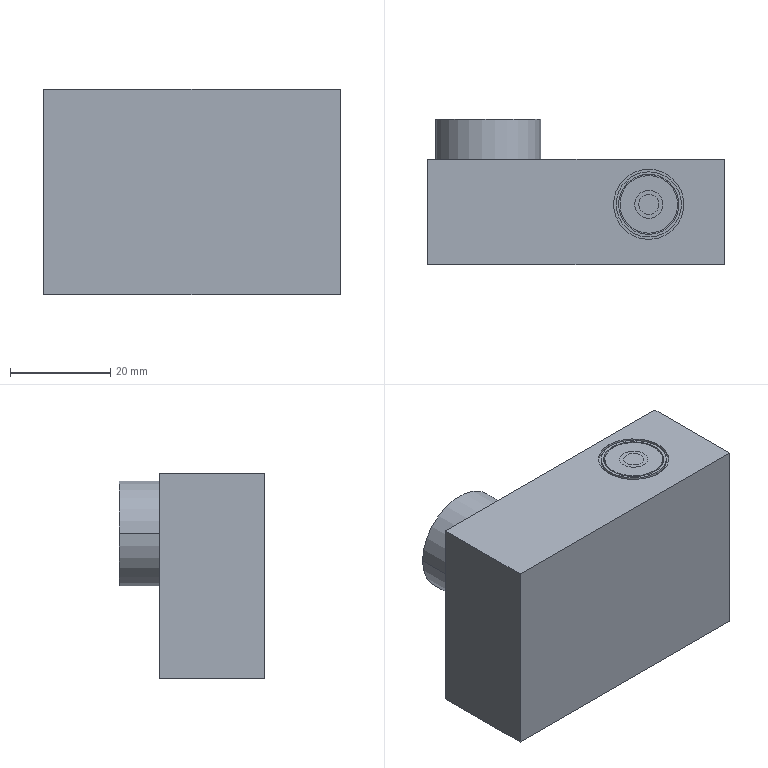Component | SolidWorks | Camera-1 | 1 solid | 38 faces | box 59 x 29 x 41 mm | volume 53051 mm3 | plane 18 | cylinder 14 | cone 4 | sphere 2 | commonest cylinder face diameters 11.5 x2 12 x2 14 x2 13 x2 17.5 x2 18.5 x2 21 x2
build123d program:
from build123d import *

# Parameters (mm, degrees)
SKETCH1_W           = 59
SKETCH1_H           = 41
BOSS_EXTRUDE1_DEPTH = 21
SKETCH5_R           = 7
SKETCH5_R_2         = 6.5
SKETCH5_R_3         = 6
SKETCH5_R_4         = 5.75
CUT_EXTRUDE1_DEPTH  = 0.5
SKETCH6_R           = 6
SKETCH6_R_2         = 5.75
CUT_EXTRUDE3_DEPTH  = 1.5


with BuildPart() as part:
    # Sketch1 → Boss-Extrude1 (new body)
    with BuildSketch(Plane.XY):
        with Locations((-17.5, -8.5)):
            Rectangle(SKETCH1_W, SKETCH1_H)
    extrude(amount=BOSS_EXTRUDE1_DEPTH)

    # Sketch4 → Revolve1 (revolve)
    with BuildSketch(Plane(origin=(0, 0, 0), x_dir=(1, 0, 0), z_dir=(0, 1, 0))):
        with BuildLine():
            Line((-10.5, -21), (-10.5, -29))
            Line((-10.5, -29), (-10, -29))
            Line((-10, -29), (-9.25, -27.5))
            Line((-9.25, -27.5), (-9.25, -26))
            Line((-9.25, -26), (-8.75, -26))
            Line((-8.75, -26), (-8.75, -27.5))
            Line((-8.75, -27.5), (-7.55, -27.5))
            Line((-7.55, -27.5), (-6.8, -26))
            ThreePointArc((-6.8, -26), (-3.716, -28.216), (0, -28.998))
            Line((0, -28.998), (0, -21))
            Line((0, -21), (-10.5, -21))
        make_face()
    revolve(axis=Axis((0, 0, 0), (0, 0, 1)))

    # Sketch5 → Cut-Extrude1 (cut)
    # profile 1 of 2: a face of its own
    with BuildSketch(Plane(origin=(0, 12, 0), x_dir=(1, 0, 0), z_dir=(0, 1, 0))):
        with Locations(Location((-32, -12, 0), (0, 0, 270))):
            Circle(SKETCH5_R)
        with Locations(Location((-32, -12, 0), (0, 0, 270))):
            Circle(SKETCH5_R_2, mode=Mode.SUBTRACT)
    # profile 2 of 2: a face of its own
    with BuildSketch(Plane(origin=(0, 12, 0), x_dir=(1, 0, 0), z_dir=(0, 1, 0))):
        with Locations(Location((-32, -12, 0), (0, 0, 270))):
            Circle(SKETCH5_R_3)
        with Locations(Location((-32, -12, 0), (0, 0, 270))):
            Circle(SKETCH5_R_4, mode=Mode.SUBTRACT)
    extrude(amount=-CUT_EXTRUDE1_DEPTH, mode=Mode.SUBTRACT)

    # Sketch6 → Cut-Extrude3 (cut)
    with BuildSketch(Plane(origin=(0, 11.5, 0), x_dir=(1, 0, 0), z_dir=(0, 1, 0))):
        with Locations(Location((-32, -12, 0), (0, 0, 270))):
            Circle(SKETCH6_R)
        with Locations(Location((-32, -12, 0), (0, 0, 270))):
            Circle(SKETCH6_R_2, mode=Mode.SUBTRACT)
    extrude(amount=-CUT_EXTRUDE3_DEPTH, mode=Mode.SUBTRACT)


solid = part.part

# Placed as in the assembly
solid = solid.moved(Location((-16.083, 97.685, 1030.6), (-90, 0, 180)))
STEP:
#1=COLOUR_RGB('',0.7922,0.8196,0.9333);
#2=FILL_AREA_STYLE_COLOUR('',#1);
#3=FILL_AREA_STYLE('',(#2));
#4=SURFACE_STYLE_FILL_AREA(#3);
#5=SURFACE_SIDE_STYLE('',(#4));
#6=SURFACE_STYLE_USAGE(.BOTH.,#5);
#7=PRESENTATION_STYLE_ASSIGNMENT((#6));
#8=CARTESIAN_POINT('',(0.6267,4.545,40.969));
#9=VERTEX_POINT('',#8);
#10=CARTESIAN_POINT('',(0.6267,4.092,40.969));
#11=VERTEX_POINT('',#10);
#12=CARTESIAN_POINT('',(0.6267,4.318,40.969));
#13=DIRECTION('',(-0.,0.,1.));
#14=DIRECTION('',(-0.,1.,0.));
#15=AXIS2_PLACEMENT_3D('',#12,#13,#14);
#16=CIRCLE('',#15,0.2264);
#17=EDGE_CURVE('',#9,#11,#16,.T.);
#18=ORIENTED_EDGE('',*,*,#17,.T.);
#19=CARTESIAN_POINT('',(0.6267,4.092,41.047));
#20=VERTEX_POINT('',#19);
#21=CARTESIAN_POINT('',(0.6267,4.092,41.028));
#22=DIRECTION('',(-0.,0.,1.));
#23=VECTOR('',#22,39.37);
#24=LINE('',#21,#23);
#25=EDGE_CURVE('',#11,#20,#24,.T.);
#26=ORIENTED_EDGE('',*,*,#25,.T.);
#27=CARTESIAN_POINT('',(0.6267,4.545,41.047));
#28=VERTEX_POINT('',#27);
#29=CARTESIAN_POINT('',(0.6267,4.318,41.047));
#30=DIRECTION('',(-0.,0.,1.));
#31=DIRECTION('',(-0.,1.,0.));
#32=AXIS2_PLACEMENT_3D('',#29,#30,#31);
#33=CIRCLE('',#32,0.2264);
#34=EDGE_CURVE('',#28,#20,#33,.T.);
#35=ORIENTED_EDGE('',*,*,#34,.F.);
#36=CARTESIAN_POINT('',(0.6267,4.545,41.028));
#37=DIRECTION('',(-0.,0.,1.));
#38=VECTOR('',#37,39.37);
#39=LINE('',#36,#38);
#40=EDGE_CURVE('',#9,#28,#39,.T.);
#41=ORIENTED_EDGE('',*,*,#40,.F.);
#42=EDGE_LOOP('',(#18,#26,#35,#41));
#43=FACE_OUTER_BOUND('',#42,.T.);
#44=CARTESIAN_POINT('',(0.6267,4.318,41.028));
#45=DIRECTION('',(-0.,0.,1.));
#46=DIRECTION('',(-0.,1.,0.));
#47=AXIS2_PLACEMENT_3D('',#44,#45,#46);
#48=CYLINDRICAL_SURFACE('',#47,0.2264);
#49=ADVANCED_FACE('',(#43),#48,.T.);
#50=CARTESIAN_POINT('',(0.6267,4.082,40.969));
#51=VERTEX_POINT('',#50);
#52=CARTESIAN_POINT('',(0.6267,4.555,40.969));
#53=VERTEX_POINT('',#52);
#54=CARTESIAN_POINT('',(0.6267,4.318,40.969));
#55=DIRECTION('',(-0.,0.,1.));
#56=DIRECTION('',(-0.,1.,0.));
#57=AXIS2_PLACEMENT_3D('',#54,#55,#56);
#58=CIRCLE('',#57,0.2362);
#59=EDGE_CURVE('',#51,#53,#58,.T.);
#60=ORIENTED_EDGE('',*,*,#59,.F.);
#61=CARTESIAN_POINT('',(0.6267,4.082,41.047));
#62=VERTEX_POINT('',#61);
#63=CARTESIAN_POINT('',(0.6267,4.082,41.028));
#64=DIRECTION('',(-0.,0.,1.));
#65=VECTOR('',#64,39.37);
#66=LINE('',#63,#65);
#67=EDGE_CURVE('',#51,#62,#66,.T.);
#68=ORIENTED_EDGE('',*,*,#67,.T.);
#69=CARTESIAN_POINT('',(0.6267,4.555,41.047));
#70=VERTEX_POINT('',#69);
#71=CARTESIAN_POINT('',(0.6267,4.318,41.047));
#72=DIRECTION('',(-0.,0.,1.));
#73=DIRECTION('',(-0.,1.,0.));
#74=AXIS2_PLACEMENT_3D('',#71,#72,#73);
#75=CIRCLE('',#74,0.2362);
#76=EDGE_CURVE('',#62,#70,#75,.T.);
#77=ORIENTED_EDGE('',*,*,#76,.T.);
#78=CARTESIAN_POINT('',(0.6267,4.555,41.028));
#79=DIRECTION('',(-0.,0.,1.));
#80=VECTOR('',#79,39.37);
#81=LINE('',#78,#80);
#82=EDGE_CURVE('',#53,#70,#81,.T.);
#83=ORIENTED_EDGE('',*,*,#82,.F.);
#84=EDGE_LOOP('',(#60,#68,#77,#83));
#85=FACE_OUTER_BOUND('',#84,.T.);
#86=CARTESIAN_POINT('',(0.6267,4.318,41.028));
#87=DIRECTION('',(-0.,0.,1.));
#88=DIRECTION('',(-0.,1.,0.));
#89=AXIS2_PLACEMENT_3D('',#86,#87,#88);
#90=CYLINDRICAL_SURFACE('',#89,0.2362);
#91=ADVANCED_FACE('',(#85),#90,.F.);
#92=CARTESIAN_POINT('',(0.6267,4.043,41.028));
#93=VERTEX_POINT('',#92);
#94=CARTESIAN_POINT('',(0.6267,4.594,41.028));
#95=VERTEX_POINT('',#94);
#96=CARTESIAN_POINT('',(0.6267,4.318,41.028));
#97=DIRECTION('',(-0.,0.,1.));
#98=DIRECTION('',(-0.,1.,0.));
#99=AXIS2_PLACEMENT_3D('',#96,#97,#98);
#100=CIRCLE('',#99,0.2756);
#101=EDGE_CURVE('',#93,#95,#100,.T.);
#102=ORIENTED_EDGE('',*,*,#101,.F.);
#103=CARTESIAN_POINT('',(0.6267,4.043,41.047));
#104=VERTEX_POINT('',#103);
#105=CARTESIAN_POINT('',(0.6267,4.043,41.028));
#106=DIRECTION('',(-0.,0.,1.));
#107=VECTOR('',#106,39.37);
#108=LINE('',#105,#107);
#109=EDGE_CURVE('',#93,#104,#108,.T.);
#110=ORIENTED_EDGE('',*,*,#109,.T.);
#111=CARTESIAN_POINT('',(0.6267,4.594,41.047));
#112=VERTEX_POINT('',#111);
#113=CARTESIAN_POINT('',(0.6267,4.318,41.047));
#114=DIRECTION('',(-0.,0.,1.));
#115=DIRECTION('',(-0.,1.,0.));
#116=AXIS2_PLACEMENT_3D('',#113,#114,#115);
#117=CIRCLE('',#116,0.2756);
#118=EDGE_CURVE('',#104,#112,#117,.T.);
#119=ORIENTED_EDGE('',*,*,#118,.T.);
#120=CARTESIAN_POINT('',(0.6267,4.594,41.028));
#121=DIRECTION('',(-0.,0.,1.));
#122=VECTOR('',#121,39.37);
#123=LINE('',#120,#122);
#124=EDGE_CURVE('',#95,#112,#123,.T.);
#125=ORIENTED_EDGE('',*,*,#124,.F.);
#126=EDGE_LOOP('',(#102,#110,#119,#125));
#127=FACE_OUTER_BOUND('',#126,.T.);
#128=CARTESIAN_POINT('',(0.6267,4.318,41.028));
#129=DIRECTION('',(-0.,0.,1.));
#130=DIRECTION('',(-0.,1.,0.));
#131=AXIS2_PLACEMENT_3D('',#128,#129,#130);
#132=CYLINDRICAL_SURFACE('',#131,0.2756);
#133=ADVANCED_FACE('',(#127),#132,.F.);
#134=CARTESIAN_POINT('',(0.6267,4.574,41.028));
#135=VERTEX_POINT('',#134);
#136=CARTESIAN_POINT('',(0.6267,4.062,41.028));
#137=VERTEX_POINT('',#136);
#138=CARTESIAN_POINT('',(0.6267,4.318,41.028));
#139=DIRECTION('',(-0.,0.,1.));
#140=DIRECTION('',(-0.,1.,0.));
#141=AXIS2_PLACEMENT_3D('',#138,#139,#140);
#142=CIRCLE('',#141,0.2559);
#143=EDGE_CURVE('',#135,#137,#142,.T.);
#144=ORIENTED_EDGE('',*,*,#143,.T.);
#145=CARTESIAN_POINT('',(0.6267,4.062,41.047));
#146=VERTEX_POINT('',#145);
#147=CARTESIAN_POINT('',(0.6267,4.062,41.028));
#148=DIRECTION('',(-0.,0.,1.));
#149=VECTOR('',#148,39.37);
#150=LINE('',#147,#149);
#151=EDGE_CURVE('',#137,#146,#150,.T.);
#152=ORIENTED_EDGE('',*,*,#151,.T.);
#153=CARTESIAN_POINT('',(0.6267,4.574,41.047));
#154=VERTEX_POINT('',#153);
#155=CARTESIAN_POINT('',(0.6267,4.318,41.047));
#156=DIRECTION('',(-0.,0.,1.));
#157=DIRECTION('',(-0.,1.,0.));
#158=AXIS2_PLACEMENT_3D('',#155,#156,#157);
#159=CIRCLE('',#158,0.2559);
#160=EDGE_CURVE('',#154,#146,#159,.T.);
#161=ORIENTED_EDGE('',*,*,#160,.F.);
#162=CARTESIAN_POINT('',(0.6267,4.574,41.028));
#163=DIRECTION('',(-0.,0.,1.));
#164=VECTOR('',#163,39.37);
#165=LINE('',#162,#164);
#166=EDGE_CURVE('',#135,#154,#165,.T.);
#167=ORIENTED_EDGE('',*,*,#166,.F.);
#168=EDGE_LOOP('',(#144,#152,#161,#167));
#169=FACE_OUTER_BOUND('',#168,.T.);
#170=CARTESIAN_POINT('',(0.6267,4.318,41.028));
#171=DIRECTION('',(-0.,0.,1.));
#172=DIRECTION('',(-0.,1.,0.));
#173=AXIS2_PLACEMENT_3D('',#170,#171,#172);
#174=CYLINDRICAL_SURFACE('',#173,0.2559);
#175=ADVANCED_FACE('',(#169),#174,.T.);
#176=CARTESIAN_POINT('',(-0.6332,4.988,40.575));
#177=VERTEX_POINT('',#176);
#178=CARTESIAN_POINT('',(-0.3655,4.869,40.575));
#179=VERTEX_POINT('',#178);
#180=CARTESIAN_POINT('',(-0.6332,4.625,40.575));
#181=DIRECTION('',(0.,-0.,-1.));
#182=DIRECTION('',(0.,1.,0.));
#183=AXIS2_PLACEMENT_3D('',#180,#181,#182);
#184=CIRCLE('',#183,0.3626);
#185=EDGE_CURVE('',#177,#179,#184,.T.);
#186=ORIENTED_EDGE('',*,*,#185,.F.);
#187=CARTESIAN_POINT('',(-0.9009,4.869,40.575));
#188=VERTEX_POINT('',#187);
#189=CARTESIAN_POINT('',(-0.6332,4.625,40.575));
#190=DIRECTION('',(0.,0.,1.));
#191=DIRECTION('',(1.,0.,0.));
#192=AXIS2_PLACEMENT_3D('',#189,#190,#191);
#193=CIRCLE('',#192,0.3626);
#194=EDGE_CURVE('',#177,#188,#193,.T.);
#195=ORIENTED_EDGE('',*,*,#194,.T.);
#196=CARTESIAN_POINT('',(-0.6332,4.869,40.575));
#197=DIRECTION('',(0.,-1.,0.));
#198=DIRECTION('',(1.,0.,0.));
#199=AXIS2_PLACEMENT_3D('',#196,#197,#198);
#200=CIRCLE('',#199,0.2677);
#201=EDGE_CURVE('',#179,#188,#200,.T.);
#202=ORIENTED_EDGE('',*,*,#201,.F.);
#203=EDGE_LOOP('',(#186,#195,#202));
#204=FACE_OUTER_BOUND('',#203,.T.);
#205=CARTESIAN_POINT('',(-0.6332,4.625,40.575));
#206=DIRECTION('',(-0.,0.,1.));
#207=DIRECTION('',(1.,0.,0.));
#208=AXIS2_PLACEMENT_3D('',#205,#206,#207);
#209=SPHERICAL_SURFACE('',#208,0.3626);
#210=ADVANCED_FACE('',(#204),#209,.T.);
#211=CARTESIAN_POINT('',(-0.6332,4.869,40.575));
#212=DIRECTION('',(0.,-1.,0.));
#213=DIRECTION('',(1.,0.,0.));
#214=AXIS2_PLACEMENT_3D('',#211,#212,#213);
#215=CIRCLE('',#214,0.2677);
#216=EDGE_CURVE('',#188,#179,#215,.T.);
#217=ORIENTED_EDGE('',*,*,#216,.T.);
#218=CARTESIAN_POINT('',(-0.3359,4.929,40.575));
#219=VERTEX_POINT('',#218);
#220=CARTESIAN_POINT('',(-0.3359,4.929,40.575));
#221=DIRECTION('',(0.4472,0.8944,0.));
#222=VECTOR('',#221,39.37);
#223=LINE('',#220,#222);
#224=EDGE_CURVE('',#179,#219,#223,.T.);
#225=ORIENTED_EDGE('',*,*,#224,.T.);
#226=CARTESIAN_POINT('',(-0.9304,4.929,40.575));
#227=VERTEX_POINT('',#226);
#228=CARTESIAN_POINT('',(-0.6332,4.929,40.575));
#229=DIRECTION('',(0.,-1.,0.));
#230=DIRECTION('',(1.,0.,0.));
#231=AXIS2_PLACEMENT_3D('',#228,#229,#230);
#232=CIRCLE('',#231,0.2972);
#233=EDGE_CURVE('',#227,#219,#232,.T.);
#234=ORIENTED_EDGE('',*,*,#233,.F.);
#235=CARTESIAN_POINT('',(-0.9304,4.929,40.575));
#236=DIRECTION('',(-0.4472,0.8944,-0.));
#237=VECTOR('',#236,39.37);
#238=LINE('',#235,#237);
#239=EDGE_CURVE('',#188,#227,#238,.T.);
#240=ORIENTED_EDGE('',*,*,#239,.F.);
#241=EDGE_LOOP('',(#217,#225,#234,#240));
#242=FACE_OUTER_BOUND('',#241,.T.);
#243=CARTESIAN_POINT('',(-0.6332,4.929,40.575));
#244=DIRECTION('',(-0.,1.,-0.));
#245=DIRECTION('',(-1.,-0.,0.));
#246=AXIS2_PLACEMENT_3D('',#243,#244,#245);
#247=CONICAL_SURFACE('',#246,0.2972,0.4636);
#248=ADVANCED_FACE('',(#242),#247,.F.);
#249=CARTESIAN_POINT('',(-0.2887,4.929,40.575));
#250=VERTEX_POINT('',#249);
#251=CARTESIAN_POINT('',(-0.9777,4.929,40.575));
#252=VERTEX_POINT('',#251);
#253=CARTESIAN_POINT('',(-0.6332,4.929,40.575));
#254=DIRECTION('',(0.,-1.,0.));
#255=DIRECTION('',(1.,0.,0.));
#256=AXIS2_PLACEMENT_3D('',#253,#254,#255);
#257=CIRCLE('',#256,0.3445);
#258=EDGE_CURVE('',#250,#252,#257,.T.);
#259=ORIENTED_EDGE('',*,*,#258,.T.);
#260=CARTESIAN_POINT('',(-0.9777,4.869,40.575));
#261=VERTEX_POINT('',#260);
#262=CARTESIAN_POINT('',(-0.9777,3.846,40.575));
#263=DIRECTION('',(0.,-1.,0.));
#264=VECTOR('',#263,39.37);
#265=LINE('',#262,#264);
#266=EDGE_CURVE('',#252,#261,#265,.T.);
#267=ORIENTED_EDGE('',*,*,#266,.T.);
#268=CARTESIAN_POINT('',(-0.2887,4.869,40.575));
#269=VERTEX_POINT('',#268);
#270=CARTESIAN_POINT('',(-0.6332,4.869,40.575));
#271=DIRECTION('',(0.,-1.,0.));
#272=DIRECTION('',(1.,0.,0.));
#273=AXIS2_PLACEMENT_3D('',#270,#271,#272);
#274=CIRCLE('',#273,0.3445);
#275=EDGE_CURVE('',#269,#261,#274,.T.);
#276=ORIENTED_EDGE('',*,*,#275,.F.);
#277=CARTESIAN_POINT('',(-0.2887,3.846,40.575));
#278=DIRECTION('',(0.,-1.,0.));
#279=VECTOR('',#278,39.37);
#280=LINE('',#277,#279);
#281=EDGE_CURVE('',#250,#269,#280,.T.);
#282=ORIENTED_EDGE('',*,*,#281,.F.);
#283=EDGE_LOOP('',(#259,#267,#276,#282));
#284=FACE_OUTER_BOUND('',#283,.T.);
#285=CARTESIAN_POINT('',(-0.6332,3.846,40.575));
#286=DIRECTION('',(0.,-1.,0.));
#287=DIRECTION('',(1.,0.,0.));
#288=AXIS2_PLACEMENT_3D('',#285,#286,#287);
#289=CYLINDRICAL_SURFACE('',#288,0.3445);
#290=ADVANCED_FACE('',(#284),#289,.T.);
#291=CARTESIAN_POINT('',(-0.9974,4.929,40.575));
#292=VERTEX_POINT('',#291);
#293=CARTESIAN_POINT('',(-0.269,4.929,40.575));
#294=VERTEX_POINT('',#293);
#295=CARTESIAN_POINT('',(-0.6332,4.929,40.575));
#296=DIRECTION('',(0.,-1.,0.));
#297=DIRECTION('',(1.,0.,0.));
#298=AXIS2_PLACEMENT_3D('',#295,#296,#297);
#299=CIRCLE('',#298,0.3642);
#300=EDGE_CURVE('',#292,#294,#299,.T.);
#301=ORIENTED_EDGE('',*,*,#300,.F.);
#302=CARTESIAN_POINT('',(-0.9974,4.869,40.575));
#303=VERTEX_POINT('',#302);
#304=CARTESIAN_POINT('',(-0.9974,3.846,40.575));
#305=DIRECTION('',(0.,-1.,0.));
#306=VECTOR('',#305,39.37);
#307=LINE('',#304,#306);
#308=EDGE_CURVE('',#292,#303,#307,.T.);
#309=ORIENTED_EDGE('',*,*,#308,.T.);
#310=CARTESIAN_POINT('',(-0.269,4.869,40.575));
#311=VERTEX_POINT('',#310);
#312=CARTESIAN_POINT('',(-0.6332,4.869,40.575));
#313=DIRECTION('',(0.,-1.,0.));
#314=DIRECTION('',(1.,0.,0.));
#315=AXIS2_PLACEMENT_3D('',#312,#313,#314);
#316=CIRCLE('',#315,0.3642);
#317=EDGE_CURVE('',#303,#311,#316,.T.);
#318=ORIENTED_EDGE('',*,*,#317,.T.);
#319=CARTESIAN_POINT('',(-0.269,3.846,40.575));
#320=DIRECTION('',(0.,-1.,0.));
#321=VECTOR('',#320,39.37);
#322=LINE('',#319,#321);
#323=EDGE_CURVE('',#294,#311,#322,.T.);
#324=ORIENTED_EDGE('',*,*,#323,.F.);
#325=EDGE_LOOP('',(#301,#309,#318,#324));
#326=FACE_OUTER_BOUND('',#325,.T.);
#327=CARTESIAN_POINT('',(-0.6332,3.846,40.575));
#328=DIRECTION('',(0.,-1.,0.));
#329=DIRECTION('',(1.,0.,0.));
#330=AXIS2_PLACEMENT_3D('',#327,#328,#329);
#331=CYLINDRICAL_SURFACE('',#330,0.3642);
#332=ADVANCED_FACE('',(#326),#331,.F.);
#333=ORIENTED_EDGE('',*,*,#300,.T.);
#334=CARTESIAN_POINT('',(-0.2395,4.988,40.575));
#335=VERTEX_POINT('',#334);
#336=CARTESIAN_POINT('',(-0.2395,4.988,40.575));
#337=DIRECTION('',(0.4472,0.8944,0.));
#338=VECTOR('',#337,39.37);
#339=LINE('',#336,#338);
#340=EDGE_CURVE('',#294,#335,#339,.T.);
#341=ORIENTED_EDGE('',*,*,#340,.T.);
#342=CARTESIAN_POINT('',(-1.027,4.988,40.575));
#343=VERTEX_POINT('',#342);
#344=CARTESIAN_POINT('',(-0.6332,4.988,40.575));
#345=DIRECTION('',(0.,-1.,0.));
#346=DIRECTION('',(1.,0.,0.));
#347=AXIS2_PLACEMENT_3D('',#344,#345,#346);
#348=CIRCLE('',#347,0.3937);
#349=EDGE_CURVE('',#343,#335,#348,.T.);
#350=ORIENTED_EDGE('',*,*,#349,.F.);
#351=CARTESIAN_POINT('',(-1.027,4.988,40.575));
#352=DIRECTION('',(-0.4472,0.8944,-0.));
#353=VECTOR('',#352,39.37);
#354=LINE('',#351,#353);
#355=EDGE_CURVE('',#292,#343,#354,.T.);
#356=ORIENTED_EDGE('',*,*,#355,.F.);
#357=EDGE_LOOP('',(#333,#341,#350,#356));
#358=FACE_OUTER_BOUND('',#357,.T.);
#359=CARTESIAN_POINT('',(-0.6332,4.988,40.575));
#360=DIRECTION('',(-0.,1.,-0.));
#361=DIRECTION('',(-1.,-0.,0.));
#362=AXIS2_PLACEMENT_3D('',#359,#360,#361);
#363=CONICAL_SURFACE('',#362,0.3937,0.4636);
#364=ADVANCED_FACE('',(#358),#363,.F.);
#365=CARTESIAN_POINT('',(-0.2198,4.988,40.575));
#366=VERTEX_POINT('',#365);
#367=CARTESIAN_POINT('',(-1.047,4.988,40.575));
#368=VERTEX_POINT('',#367);
#369=CARTESIAN_POINT('',(-0.6332,4.988,40.575));
#370=DIRECTION('',(0.,-1.,0.));
#371=DIRECTION('',(1.,0.,0.));
#372=AXIS2_PLACEMENT_3D('',#369,#370,#371);
#373=CIRCLE('',#372,0.4134);
#374=EDGE_CURVE('',#366,#368,#373,.T.);
#375=ORIENTED_EDGE('',*,*,#374,.T.);
#376=CARTESIAN_POINT('',(-1.047,4.673,40.575));
#377=VERTEX_POINT('',#376);
#378=CARTESIAN_POINT('',(-1.047,3.846,40.575));
#379=DIRECTION('',(0.,-1.,0.));
#380=VECTOR('',#379,39.37);
#381=LINE('',#378,#380);
#382=EDGE_CURVE('',#368,#377,#381,.T.);
#383=ORIENTED_EDGE('',*,*,#382,.T.);
#384=CARTESIAN_POINT('',(-0.2198,4.673,40.575));
#385=VERTEX_POINT('',#384);
#386=CARTESIAN_POINT('',(-0.6332,4.673,40.575));
#387=DIRECTION('',(-0.,1.,-0.));
#388=DIRECTION('',(-1.,-0.,0.));
#389=AXIS2_PLACEMENT_3D('',#386,#387,#388);
#390=CIRCLE('',#389,0.4134);
#391=EDGE_CURVE('',#377,#385,#390,.T.);
#392=ORIENTED_EDGE('',*,*,#391,.T.);
#393=CARTESIAN_POINT('',(-0.2198,3.846,40.575));
#394=DIRECTION('',(0.,-1.,0.));
#395=VECTOR('',#394,39.37);
#396=LINE('',#393,#395);
#397=EDGE_CURVE('',#366,#385,#396,.T.);
#398=ORIENTED_EDGE('',*,*,#397,.F.);
#399=EDGE_LOOP('',(#375,#383,#392,#398));
#400=FACE_OUTER_BOUND('',#399,.T.);
#401=CARTESIAN_POINT('',(-0.6332,3.846,40.575));
#402=DIRECTION('',(0.,-1.,0.));
#403=DIRECTION('',(1.,0.,0.));
#404=AXIS2_PLACEMENT_3D('',#401,#402,#403);
#405=CYLINDRICAL_SURFACE('',#404,0.4134);
#406=ADVANCED_FACE('',(#400),#405,.T.);
#407=CARTESIAN_POINT('',(0.5479,4.673,39.827));
#408=VERTEX_POINT('',#407);
#409=CARTESIAN_POINT('',(0.9416,4.673,39.827));
#410=VERTEX_POINT('',#409);
#411=CARTESIAN_POINT('',(0.7448,4.673,39.827));
#412=DIRECTION('',(0.,-1.,0.));
#413=DIRECTION('',(-1.,-0.,0.));
#414=AXIS2_PLACEMENT_3D('',#411,#412,#413);
#415=CIRCLE('',#414,0.1969);
#416=EDGE_CURVE('',#408,#410,#415,.T.);
#417=ORIENTED_EDGE('',*,*,#416,.F.);
#418=CARTESIAN_POINT('',(0.7448,4.673,39.827));
#419=DIRECTION('',(0.,-1.,0.));
#420=DIRECTION('',(-1.,-0.,0.));
#421=AXIS2_PLACEMENT_3D('',#418,#419,#420);
#422=CIRCLE('',#421,0.1969);
#423=EDGE_CURVE('',#410,#408,#422,.T.);
#424=ORIENTED_EDGE('',*,*,#423,.F.);
#425=EDGE_LOOP('',(#417,#424));
#426=FACE_OUTER_BOUND('',#425,.T.);
#427=CARTESIAN_POINT('',(0.7349,4.673,39.978));
#428=VERTEX_POINT('',#427);
#429=CARTESIAN_POINT('',(0.7349,4.673,39.86));
#430=VERTEX_POINT('',#429);
#431=CARTESIAN_POINT('',(0.7349,4.673,40.575));
#432=DIRECTION('',(0.,-0.,-1.));
#433=VECTOR('',#432,39.37);
#434=LINE('',#431,#433);
#435=EDGE_CURVE('',#428,#430,#434,.T.);
#436=ORIENTED_EDGE('',*,*,#435,.T.);
#437=CARTESIAN_POINT('',(0.7546,4.673,39.86));
#438=VERTEX_POINT('',#437);
#439=CARTESIAN_POINT('',(0.7448,4.673,39.86));
#440=DIRECTION('',(0.,-1.,0.));
#441=DIRECTION('',(-1.,0.,0.));
#442=AXIS2_PLACEMENT_3D('',#439,#440,#441);
#443=CIRCLE('',#442,0.009843);
#444=EDGE_CURVE('',#430,#438,#443,.T.);
#445=ORIENTED_EDGE('',*,*,#444,.T.);
#446=CARTESIAN_POINT('',(0.7546,4.673,39.978));
#447=VERTEX_POINT('',#446);
#448=CARTESIAN_POINT('',(0.7546,4.673,40.575));
#449=DIRECTION('',(-0.,0.,1.));
#450=VECTOR('',#449,39.37);
#451=LINE('',#448,#450);
#452=EDGE_CURVE('',#438,#447,#451,.T.);
#453=ORIENTED_EDGE('',*,*,#452,.T.);
#454=CARTESIAN_POINT('',(0.7448,4.673,39.978));
#455=DIRECTION('',(0.,-1.,0.));
#456=DIRECTION('',(-1.,0.,0.));
#457=AXIS2_PLACEMENT_3D('',#454,#455,#456);
#458=CIRCLE('',#457,0.009843);
#459=EDGE_CURVE('',#447,#428,#458,.T.);
#460=ORIENTED_EDGE('',*,*,#459,.T.);
#461=EDGE_LOOP('',(#436,#445,#453,#460));
#462=FACE_BOUND('',#461,.T.);
#463=CARTESIAN_POINT('',(0.6628,4.673,39.928));
#464=VERTEX_POINT('',#463);
#465=CARTESIAN_POINT('',(0.8268,4.673,39.928));
#466=VERTEX_POINT('',#465);
#467=CARTESIAN_POINT('',(0.7448,4.673,39.815));
#468=DIRECTION('',(0.,-1.,0.));
#469=DIRECTION('',(-1.,-0.,-0.));
#470=AXIS2_PLACEMENT_3D('',#467,#468,#469);
#471=CIRCLE('',#470,0.139);
#472=EDGE_CURVE('',#464,#466,#471,.T.);
#473=ORIENTED_EDGE('',*,*,#472,.T.);
#474=CARTESIAN_POINT('',(0.8138,4.673,39.91));
#475=VERTEX_POINT('',#474);
#476=CARTESIAN_POINT('',(0.8203,4.673,39.919));
#477=DIRECTION('',(0.,-1.,0.));
#478=DIRECTION('',(-1.,0.,0.));
#479=AXIS2_PLACEMENT_3D('',#476,#477,#478);
#480=CIRCLE('',#479,0.01102);
#481=EDGE_CURVE('',#466,#475,#480,.T.);
#482=ORIENTED_EDGE('',*,*,#481,.T.);
#483=CARTESIAN_POINT('',(0.6758,4.673,39.91));
#484=VERTEX_POINT('',#483);
#485=CARTESIAN_POINT('',(0.7448,4.673,39.815));
#486=DIRECTION('',(-0.,1.,-0.));
#487=DIRECTION('',(-1.,-0.,0.));
#488=AXIS2_PLACEMENT_3D('',#485,#486,#487);
#489=CIRCLE('',#488,0.1169);
#490=EDGE_CURVE('',#475,#484,#489,.T.);
#491=ORIENTED_EDGE('',*,*,#490,.T.);
#492=CARTESIAN_POINT('',(0.6693,4.673,39.919));
#493=DIRECTION('',(0.,-1.,0.));
#494=DIRECTION('',(-1.,0.,0.));
#495=AXIS2_PLACEMENT_3D('',#492,#493,#494);
#496=CIRCLE('',#495,0.01102);
#497=EDGE_CURVE('',#484,#464,#496,.T.);
#498=ORIENTED_EDGE('',*,*,#497,.T.);
#499=EDGE_LOOP('',(#473,#482,#491,#498));
#500=FACE_BOUND('',#499,.T.);
#501=CARTESIAN_POINT('',(-0.6332,4.673,40.575));
#502=DIRECTION('',(-0.,1.,-0.));
#503=DIRECTION('',(-1.,-0.,-0.));
#504=AXIS2_PLACEMENT_3D('',#501,#502,#503);
#505=PLANE('',#504);
#506=ADVANCED_FACE('',(#426,#462,#500),#505,.T.);
#507=ORIENTED_EDGE('',*,*,#481,.F.);
#508=ORIENTED_EDGE('',*,*,#472,.F.);
#509=ORIENTED_EDGE('',*,*,#497,.F.);
#510=ORIENTED_EDGE('',*,*,#490,.F.);
#511=EDGE_LOOP('',(#507,#508,#509,#510));
#512=FACE_OUTER_BOUND('',#511,.T.);
#513=CARTESIAN_POINT('',(-0.6332,4.673,40.575));
#514=DIRECTION('',(-0.,1.,-0.));
#515=DIRECTION('',(-1.,-0.,-0.));
#516=AXIS2_PLACEMENT_3D('',#513,#514,#515);
#517=PLANE('',#516);
#518=ADVANCED_FACE('',(#512),#517,.T.);
#519=CARTESIAN_POINT('',(1.217,4.673,41.047));
#520=VERTEX_POINT('',#519);
#521=CARTESIAN_POINT('',(1.217,4.673,39.433));
#522=VERTEX_POINT('',#521);
#523=CARTESIAN_POINT('',(1.217,4.673,41.047));
#524=DIRECTION('',(-0.,-0.,-1.));
#525=VECTOR('',#524,39.37);
#526=LINE('',#523,#525);
#527=EDGE_CURVE('',#520,#522,#526,.T.);
#528=ORIENTED_EDGE('',*,*,#527,.T.);
#529=CARTESIAN_POINT('',(-1.106,4.673,39.433));
#530=VERTEX_POINT('',#529);
#531=CARTESIAN_POINT('',(1.217,4.673,39.433));
#532=DIRECTION('',(-1.,-0.,-0.));
#533=VECTOR('',#532,39.37);
#534=LINE('',#531,#533);
#535=EDGE_CURVE('',#522,#530,#534,.T.);
#536=ORIENTED_EDGE('',*,*,#535,.T.);
#537=CARTESIAN_POINT('',(-1.106,4.673,41.047));
#538=VERTEX_POINT('',#537);
#539=CARTESIAN_POINT('',(-1.106,4.673,41.047));
#540=DIRECTION('',(0.,0.,1.));
#541=VECTOR('',#540,39.37);
#542=LINE('',#539,#541);
#543=EDGE_CURVE('',#530,#538,#542,.T.);
#544=ORIENTED_EDGE('',*,*,#543,.T.);
#545=CARTESIAN_POINT('',(1.217,4.673,41.047));
#546=DIRECTION('',(1.,0.,0.));
#547=VECTOR('',#546,39.37);
#548=LINE('',#545,#547);
#549=EDGE_CURVE('',#538,#520,#548,.T.);
#550=ORIENTED_EDGE('',*,*,#549,.T.);
#551=EDGE_LOOP('',(#528,#536,#544,#550));
#552=FACE_OUTER_BOUND('',#551,.T.);
#553=CARTESIAN_POINT('',(-0.6332,4.673,40.575));
#554=DIRECTION('',(-0.,1.,-0.));
#555=DIRECTION('',(-1.,-0.,0.));
#556=AXIS2_PLACEMENT_3D('',#553,#554,#555);
#557=CIRCLE('',#556,0.4134);
#558=EDGE_CURVE('',#385,#377,#557,.T.);
#559=ORIENTED_EDGE('',*,*,#558,.F.);
#560=ORIENTED_EDGE('',*,*,#391,.F.);
#561=EDGE_LOOP('',(#559,#560));
#562=FACE_BOUND('',#561,.T.);
#563=ORIENTED_EDGE('',*,*,#416,.T.);
#564=ORIENTED_EDGE('',*,*,#423,.T.);
#565=EDGE_LOOP('',(#563,#564));
#566=FACE_BOUND('',#565,.T.);
#567=CARTESIAN_POINT('',(-0.6332,4.673,40.575));
#568=DIRECTION('',(-0.,1.,-0.));
#569=DIRECTION('',(-1.,-0.,-0.));
#570=AXIS2_PLACEMENT_3D('',#567,#568,#569);
#571=PLANE('',#570);
#572=ADVANCED_FACE('',(#552,#562,#566),#571,.T.);
#573=CARTESIAN_POINT('',(0.6267,4.209,41.047));
#574=VERTEX_POINT('',#573);
#575=CARTESIAN_POINT('',(0.6267,4.428,41.047));
#576=VERTEX_POINT('',#575);
#577=CARTESIAN_POINT('',(0.6267,4.318,41.047));
#578=DIRECTION('',(-0.,0.,1.));
#579=DIRECTION('',(0.,-1.,0.));
#580=AXIS2_PLACEMENT_3D('',#577,#578,#579);
#581=CIRCLE('',#580,0.1094);
#582=EDGE_CURVE('',#574,#576,#581,.T.);
#583=ORIENTED_EDGE('',*,*,#582,.T.);
#584=CARTESIAN_POINT('',(0.6267,4.318,41.047));
#585=DIRECTION('',(-0.,0.,1.));
#586=DIRECTION('',(0.,-1.,0.));
#587=AXIS2_PLACEMENT_3D('',#584,#585,#586);
#588=CIRCLE('',#587,0.1094);
#589=EDGE_CURVE('',#576,#574,#588,.T.);
#590=ORIENTED_EDGE('',*,*,#589,.T.);
#591=EDGE_LOOP('',(#583,#590));
#592=FACE_OUTER_BOUND('',#591,.T.);
#593=CARTESIAN_POINT('',(0.6267,4.24,41.047));
#594=VERTEX_POINT('',#593);
#595=CARTESIAN_POINT('',(0.6267,4.397,41.047));
#596=VERTEX_POINT('',#595);
#597=CARTESIAN_POINT('',(0.6267,4.318,41.047));
#598=DIRECTION('',(-0.,0.,1.));
#599=DIRECTION('',(0.,-1.,0.));
#600=AXIS2_PLACEMENT_3D('',#597,#598,#599);
#601=CIRCLE('',#600,0.07874);
#602=EDGE_CURVE('',#594,#596,#601,.T.);
#603=ORIENTED_EDGE('',*,*,#602,.F.);
#604=CARTESIAN_POINT('',(0.6267,4.318,41.047));
#605=DIRECTION('',(-0.,0.,1.));
#606=DIRECTION('',(0.,-1.,0.));
#607=AXIS2_PLACEMENT_3D('',#604,#605,#606);
#608=CIRCLE('',#607,0.07874);
#609=EDGE_CURVE('',#596,#594,#608,.T.);
#610=ORIENTED_EDGE('',*,*,#609,.F.);
#611=EDGE_LOOP('',(#603,#610));
#612=FACE_BOUND('',#611,.T.);
#613=CARTESIAN_POINT('',(1.217,4.673,41.047));
#614=DIRECTION('',(0.,-0.,-1.));
#615=DIRECTION('',(0.,-1.,0.));
#616=AXIS2_PLACEMENT_3D('',#613,#614,#615);
#617=PLANE('',#616);
#618=ADVANCED_FACE('',(#592,#612),#617,.F.);
#619=ORIENTED_EDGE('',*,*,#34,.T.);
#620=CARTESIAN_POINT('',(0.6267,4.318,41.047));
#621=DIRECTION('',(-0.,0.,1.));
#622=DIRECTION('',(-0.,1.,0.));
#623=AXIS2_PLACEMENT_3D('',#620,#621,#622);
#624=CIRCLE('',#623,0.2264);
#625=EDGE_CURVE('',#20,#28,#624,.T.);
#626=ORIENTED_EDGE('',*,*,#625,.T.);
#627=EDGE_LOOP('',(#619,#626));
#628=FACE_OUTER_BOUND('',#627,.T.);
#629=ORIENTED_EDGE('',*,*,#582,.F.);
#630=ORIENTED_EDGE('',*,*,#589,.F.);
#631=EDGE_LOOP('',(#629,#630));
#632=FACE_BOUND('',#631,.T.);
#633=CARTESIAN_POINT('',(1.217,4.673,41.047));
#634=DIRECTION('',(0.,-0.,-1.));
#635=DIRECTION('',(0.,-1.,0.));
#636=AXIS2_PLACEMENT_3D('',#633,#634,#635);
#637=PLANE('',#636);
#638=ADVANCED_FACE('',(#628,#632),#637,.F.);
#639=CARTESIAN_POINT('',(1.217,3.846,41.047));
#640=VERTEX_POINT('',#639);
#641=CARTESIAN_POINT('',(1.217,3.846,39.433));
#642=VERTEX_POINT('',#641);
#643=CARTESIAN_POINT('',(1.217,3.846,41.047));
#644=DIRECTION('',(-0.,-0.,-1.));
#645=VECTOR('',#644,39.37);
#646=LINE('',#643,#645);
#647=EDGE_CURVE('',#640,#642,#646,.T.);
#648=ORIENTED_EDGE('',*,*,#647,.T.);
#649=CARTESIAN_POINT('',(1.217,4.673,39.433));
#650=DIRECTION('',(0.,-1.,0.));
#651=VECTOR('',#650,39.37);
#652=LINE('',#649,#651);
#653=EDGE_CURVE('',#522,#642,#652,.T.);
#654=ORIENTED_EDGE('',*,*,#653,.F.);
#655=ORIENTED_EDGE('',*,*,#527,.F.);
#656=CARTESIAN_POINT('',(1.217,4.673,41.047));
#657=DIRECTION('',(0.,-1.,0.));
#658=VECTOR('',#657,39.37);
#659=LINE('',#656,#658);
#660=EDGE_CURVE('',#520,#640,#659,.T.);
#661=ORIENTED_EDGE('',*,*,#660,.T.);
#662=EDGE_LOOP('',(#648,#654,#655,#661));
#663=FACE_OUTER_BOUND('',#662,.T.);
#664=CARTESIAN_POINT('',(1.217,4.673,41.047));
#665=DIRECTION('',(-1.,-0.,0.));
#666=DIRECTION('',(0.,0.,1.));
#667=AXIS2_PLACEMENT_3D('',#664,#665,#666);
#668=PLANE('',#667);
#669=ADVANCED_FACE('',(#663),#668,.F.);
#670=CARTESIAN_POINT('',(-1.106,3.846,39.433));
#671=VERTEX_POINT('',#670);
#672=CARTESIAN_POINT('',(1.217,3.846,39.433));
#673=DIRECTION('',(-1.,-0.,-0.));
#674=VECTOR('',#673,39.37);
#675=LINE('',#672,#674);
#676=EDGE_CURVE('',#642,#671,#675,.T.);
#677=ORIENTED_EDGE('',*,*,#676,.T.);
#678=CARTESIAN_POINT('',(-1.106,4.673,39.433));
#679=DIRECTION('',(0.,-1.,0.));
#680=VECTOR('',#679,39.37);
#681=LINE('',#678,#680);
#682=EDGE_CURVE('',#530,#671,#681,.T.);
#683=ORIENTED_EDGE('',*,*,#682,.F.);
#684=ORIENTED_EDGE('',*,*,#535,.F.);
#685=ORIENTED_EDGE('',*,*,#653,.T.);
#686=EDGE_LOOP('',(#677,#683,#684,#685));
#687=FACE_OUTER_BOUND('',#686,.T.);
#688=CARTESIAN_POINT('',(1.217,4.673,39.433));
#689=DIRECTION('',(-0.,0.,1.));
#690=DIRECTION('',(-0.,1.,-0.));
#691=AXIS2_PLACEMENT_3D('',#688,#689,#690);
#692=PLANE('',#691);
#693=ADVANCED_FACE('',(#687),#692,.F.);
#694=CARTESIAN_POINT('',(-1.106,3.846,41.047));
#695=VERTEX_POINT('',#694);
#696=CARTESIAN_POINT('',(-1.106,3.846,41.047));
#697=DIRECTION('',(0.,0.,1.));
#698=VECTOR('',#697,39.37);
#699=LINE('',#696,#698);
#700=EDGE_CURVE('',#671,#695,#699,.T.);
#701=ORIENTED_EDGE('',*,*,#700,.T.);
#702=CARTESIAN_POINT('',(-1.106,4.673,41.047));
#703=DIRECTION('',(0.,-1.,0.));
#704=VECTOR('',#703,39.37);
#705=LINE('',#702,#704);
#706=EDGE_CURVE('',#538,#695,#705,.T.);
#707=ORIENTED_EDGE('',*,*,#706,.F.);
#708=ORIENTED_EDGE('',*,*,#543,.F.);
#709=ORIENTED_EDGE('',*,*,#682,.T.);
#710=EDGE_LOOP('',(#701,#707,#708,#709));
#711=FACE_OUTER_BOUND('',#710,.T.);
#712=CARTESIAN_POINT('',(-1.106,4.673,41.047));
#713=DIRECTION('',(1.,0.,-0.));
#714=DIRECTION('',(-0.,-0.,-1.));
#715=AXIS2_PLACEMENT_3D('',#712,#713,#714);
#716=PLANE('',#715);
#717=ADVANCED_FACE('',(#711),#716,.F.);
#718=CARTESIAN_POINT('',(0.6267,4.318,41.047));
#719=DIRECTION('',(-0.,0.,1.));
#720=DIRECTION('',(-0.,1.,0.));
#721=AXIS2_PLACEMENT_3D('',#718,#719,#720);
#722=CIRCLE('',#721,0.2756);
#723=EDGE_CURVE('',#112,#104,#722,.T.);
#724=ORIENTED_EDGE('',*,*,#723,.F.);
#725=ORIENTED_EDGE('',*,*,#118,.F.);
#726=EDGE_LOOP('',(#724,#725));
#727=FACE_BOUND('',#726,.T.);
#728=CARTESIAN_POINT('',(1.217,3.846,41.047));
#729=DIRECTION('',(1.,0.,0.));
#730=VECTOR('',#729,39.37);
#731=LINE('',#728,#730);
#732=EDGE_CURVE('',#695,#640,#731,.T.);
#733=ORIENTED_EDGE('',*,*,#732,.T.);
#734=ORIENTED_EDGE('',*,*,#660,.F.);
#735=ORIENTED_EDGE('',*,*,#549,.F.);
#736=ORIENTED_EDGE('',*,*,#706,.T.);
#737=EDGE_LOOP('',(#733,#734,#735,#736));
#738=FACE_OUTER_BOUND('',#737,.T.);
#739=CARTESIAN_POINT('',(1.217,4.673,41.047));
#740=DIRECTION('',(0.,-0.,-1.));
#741=DIRECTION('',(0.,-1.,0.));
#742=AXIS2_PLACEMENT_3D('',#739,#740,#741);
#743=PLANE('',#742);
#744=ADVANCED_FACE('',(#727,#738),#743,.F.);
#745=ORIENTED_EDGE('',*,*,#444,.F.);
#746=ORIENTED_EDGE('',*,*,#435,.F.);
#747=ORIENTED_EDGE('',*,*,#459,.F.);
#748=ORIENTED_EDGE('',*,*,#452,.F.);
#749=EDGE_LOOP('',(#745,#746,#747,#748));
#750=FACE_OUTER_BOUND('',#749,.T.);
#751=CARTESIAN_POINT('',(-0.6332,4.673,40.575));
#752=DIRECTION('',(-0.,1.,-0.));
#753=DIRECTION('',(-1.,-0.,-0.));
#754=AXIS2_PLACEMENT_3D('',#751,#752,#753);
#755=PLANE('',#754);
#756=ADVANCED_FACE('',(#750),#755,.T.);
#757=ORIENTED_EDGE('',*,*,#647,.F.);
#758=ORIENTED_EDGE('',*,*,#732,.F.);
#759=ORIENTED_EDGE('',*,*,#700,.F.);
#760=ORIENTED_EDGE('',*,*,#676,.F.);
#761=EDGE_LOOP('',(#757,#758,#759,#760));
#762=FACE_OUTER_BOUND('',#761,.T.);
#763=CARTESIAN_POINT('',(-0.6332,3.846,40.575));
#764=DIRECTION('',(-0.,1.,-0.));
#765=DIRECTION('',(-1.,-0.,-0.));
#766=AXIS2_PLACEMENT_3D('',#763,#764,#765);
#767=PLANE('',#766);
#768=ADVANCED_FACE('',(#762),#767,.F.);
#769=ORIENTED_EDGE('',*,*,#382,.F.);
#770=CARTESIAN_POINT('',(-0.6332,4.988,40.575));
#771=DIRECTION('',(0.,-1.,0.));
#772=DIRECTION('',(1.,0.,0.));
#773=AXIS2_PLACEMENT_3D('',#770,#771,#772);
#774=CIRCLE('',#773,0.4134);
#775=EDGE_CURVE('',#368,#366,#774,.T.);
#776=ORIENTED_EDGE('',*,*,#775,.T.);
#777=ORIENTED_EDGE('',*,*,#397,.T.);
#778=ORIENTED_EDGE('',*,*,#558,.T.);
#779=EDGE_LOOP('',(#769,#776,#777,#778));
#780=FACE_OUTER_BOUND('',#779,.T.);
#781=CARTESIAN_POINT('',(-0.6332,3.846,40.575));
#782=DIRECTION('',(0.,-1.,0.));
#783=DIRECTION('',(1.,0.,0.));
#784=AXIS2_PLACEMENT_3D('',#781,#782,#783);
#785=CYLINDRICAL_SURFACE('',#784,0.4134);
#786=ADVANCED_FACE('',(#780),#785,.T.);
#787=ORIENTED_EDGE('',*,*,#349,.T.);
#788=CARTESIAN_POINT('',(-0.6332,4.988,40.575));
#789=DIRECTION('',(0.,-1.,0.));
#790=DIRECTION('',(1.,0.,0.));
#791=AXIS2_PLACEMENT_3D('',#788,#789,#790);
#792=CIRCLE('',#791,0.3937);
#793=EDGE_CURVE('',#335,#343,#792,.T.);
#794=ORIENTED_EDGE('',*,*,#793,.T.);
#795=EDGE_LOOP('',(#787,#794));
#796=FACE_BOUND('',#795,.T.);
#797=ORIENTED_EDGE('',*,*,#374,.F.);
#798=ORIENTED_EDGE('',*,*,#775,.F.);
#799=EDGE_LOOP('',(#797,#798));
#800=FACE_OUTER_BOUND('',#799,.T.);
#801=CARTESIAN_POINT('',(-0.2198,4.988,40.575));
#802=DIRECTION('',(-0.,1.,-0.));
#803=DIRECTION('',(-1.,-0.,-0.));
#804=AXIS2_PLACEMENT_3D('',#801,#802,#803);
#805=PLANE('',#804);
#806=ADVANCED_FACE('',(#796,#800),#805,.T.);
#807=ORIENTED_EDGE('',*,*,#340,.F.);
#808=CARTESIAN_POINT('',(-0.6332,4.929,40.575));
#809=DIRECTION('',(0.,-1.,0.));
#810=DIRECTION('',(1.,0.,0.));
#811=AXIS2_PLACEMENT_3D('',#808,#809,#810);
#812=CIRCLE('',#811,0.3642);
#813=EDGE_CURVE('',#294,#292,#812,.T.);
#814=ORIENTED_EDGE('',*,*,#813,.T.);
#815=ORIENTED_EDGE('',*,*,#355,.T.);
#816=ORIENTED_EDGE('',*,*,#793,.F.);
#817=EDGE_LOOP('',(#807,#814,#815,#816));
#818=FACE_OUTER_BOUND('',#817,.T.);
#819=CARTESIAN_POINT('',(-0.6332,4.988,40.575));
#820=DIRECTION('',(-0.,1.,-0.));
#821=DIRECTION('',(-1.,-0.,0.));
#822=AXIS2_PLACEMENT_3D('',#819,#820,#821);
#823=CONICAL_SURFACE('',#822,0.3937,0.4636);
#824=ADVANCED_FACE('',(#818),#823,.F.);
#825=ORIENTED_EDGE('',*,*,#308,.F.);
#826=ORIENTED_EDGE('',*,*,#813,.F.);
#827=ORIENTED_EDGE('',*,*,#323,.T.);
#828=CARTESIAN_POINT('',(-0.6332,4.869,40.575));
#829=DIRECTION('',(0.,-1.,0.));
#830=DIRECTION('',(1.,0.,0.));
#831=AXIS2_PLACEMENT_3D('',#828,#829,#830);
#832=CIRCLE('',#831,0.3642);
#833=EDGE_CURVE('',#311,#303,#832,.T.);
#834=ORIENTED_EDGE('',*,*,#833,.T.);
#835=EDGE_LOOP('',(#825,#826,#827,#834));
#836=FACE_OUTER_BOUND('',#835,.T.);
#837=CARTESIAN_POINT('',(-0.6332,3.846,40.575));
#838=DIRECTION('',(0.,-1.,0.));
#839=DIRECTION('',(1.,0.,0.));
#840=AXIS2_PLACEMENT_3D('',#837,#838,#839);
#841=CYLINDRICAL_SURFACE('',#840,0.3642);
#842=ADVANCED_FACE('',(#836),#841,.F.);
#843=ORIENTED_EDGE('',*,*,#275,.T.);
#844=CARTESIAN_POINT('',(-0.6332,4.869,40.575));
#845=DIRECTION('',(0.,-1.,0.));
#846=DIRECTION('',(1.,0.,0.));
#847=AXIS2_PLACEMENT_3D('',#844,#845,#846);
#848=CIRCLE('',#847,0.3445);
#849=EDGE_CURVE('',#261,#269,#848,.T.);
#850=ORIENTED_EDGE('',*,*,#849,.T.);
#851=EDGE_LOOP('',(#843,#850));
#852=FACE_BOUND('',#851,.T.);
#853=ORIENTED_EDGE('',*,*,#833,.F.);
#854=ORIENTED_EDGE('',*,*,#317,.F.);
#855=EDGE_LOOP('',(#853,#854));
#856=FACE_OUTER_BOUND('',#855,.T.);
#857=CARTESIAN_POINT('',(-0.269,4.869,40.575));
#858=DIRECTION('',(-0.,1.,-0.));
#859=DIRECTION('',(-1.,-0.,-0.));
#860=AXIS2_PLACEMENT_3D('',#857,#858,#859);
#861=PLANE('',#860);
#862=ADVANCED_FACE('',(#852,#856),#861,.T.);
#863=ORIENTED_EDGE('',*,*,#266,.F.);
#864=CARTESIAN_POINT('',(-0.6332,4.929,40.575));
#865=DIRECTION('',(0.,-1.,0.));
#866=DIRECTION('',(1.,0.,0.));
#867=AXIS2_PLACEMENT_3D('',#864,#865,#866);
#868=CIRCLE('',#867,0.3445);
#869=EDGE_CURVE('',#252,#250,#868,.T.);
#870=ORIENTED_EDGE('',*,*,#869,.T.);
#871=ORIENTED_EDGE('',*,*,#281,.T.);
#872=ORIENTED_EDGE('',*,*,#849,.F.);
#873=EDGE_LOOP('',(#863,#870,#871,#872));
#874=FACE_OUTER_BOUND('',#873,.T.);
#875=CARTESIAN_POINT('',(-0.6332,3.846,40.575));
#876=DIRECTION('',(0.,-1.,0.));
#877=DIRECTION('',(1.,0.,0.));
#878=AXIS2_PLACEMENT_3D('',#875,#876,#877);
#879=CYLINDRICAL_SURFACE('',#878,0.3445);
#880=ADVANCED_FACE('',(#874),#879,.T.);
#881=ORIENTED_EDGE('',*,*,#233,.T.);
#882=CARTESIAN_POINT('',(-0.6332,4.929,40.575));
#883=DIRECTION('',(0.,-1.,0.));
#884=DIRECTION('',(1.,0.,0.));
#885=AXIS2_PLACEMENT_3D('',#882,#883,#884);
#886=CIRCLE('',#885,0.2972);
#887=EDGE_CURVE('',#219,#227,#886,.T.);
#888=ORIENTED_EDGE('',*,*,#887,.T.);
#889=EDGE_LOOP('',(#881,#888));
#890=FACE_BOUND('',#889,.T.);
#891=ORIENTED_EDGE('',*,*,#258,.F.);
#892=ORIENTED_EDGE('',*,*,#869,.F.);
#893=EDGE_LOOP('',(#891,#892));
#894=FACE_OUTER_BOUND('',#893,.T.);
#895=CARTESIAN_POINT('',(-0.2887,4.929,40.575));
#896=DIRECTION('',(-0.,1.,-0.));
#897=DIRECTION('',(-1.,-0.,-0.));
#898=AXIS2_PLACEMENT_3D('',#895,#896,#897);
#899=PLANE('',#898);
#900=ADVANCED_FACE('',(#890,#894),#899,.T.);
#901=ORIENTED_EDGE('',*,*,#224,.F.);
#902=ORIENTED_EDGE('',*,*,#201,.T.);
#903=ORIENTED_EDGE('',*,*,#239,.T.);
#904=ORIENTED_EDGE('',*,*,#887,.F.);
#905=EDGE_LOOP('',(#901,#902,#903,#904));
#906=FACE_OUTER_BOUND('',#905,.T.);
#907=CARTESIAN_POINT('',(-0.6332,4.929,40.575));
#908=DIRECTION('',(-0.,1.,-0.));
#909=DIRECTION('',(-1.,-0.,0.));
#910=AXIS2_PLACEMENT_3D('',#907,#908,#909);
#911=CONICAL_SURFACE('',#910,0.2972,0.4636);
#912=ADVANCED_FACE('',(#906),#911,.F.);
#913=ORIENTED_EDGE('',*,*,#194,.F.);
#914=ORIENTED_EDGE('',*,*,#185,.T.);
#915=ORIENTED_EDGE('',*,*,#216,.F.);
#916=EDGE_LOOP('',(#913,#914,#915));
#917=FACE_OUTER_BOUND('',#916,.T.);
#918=CARTESIAN_POINT('',(-0.6332,4.625,40.575));
#919=DIRECTION('',(-0.,0.,1.));
#920=DIRECTION('',(1.,0.,0.));
#921=AXIS2_PLACEMENT_3D('',#918,#919,#920);
#922=SPHERICAL_SURFACE('',#921,0.3626);
#923=ADVANCED_FACE('',(#917),#922,.T.);
#924=ORIENTED_EDGE('',*,*,#151,.F.);
#925=CARTESIAN_POINT('',(0.6267,4.318,41.028));
#926=DIRECTION('',(-0.,0.,1.));
#927=DIRECTION('',(-0.,1.,0.));
#928=AXIS2_PLACEMENT_3D('',#925,#926,#927);
#929=CIRCLE('',#928,0.2559);
#930=EDGE_CURVE('',#137,#135,#929,.T.);
#931=ORIENTED_EDGE('',*,*,#930,.T.);
#932=ORIENTED_EDGE('',*,*,#166,.T.);
#933=CARTESIAN_POINT('',(0.6267,4.318,41.047));
#934=DIRECTION('',(-0.,0.,1.));
#935=DIRECTION('',(-0.,1.,0.));
#936=AXIS2_PLACEMENT_3D('',#933,#934,#935);
#937=CIRCLE('',#936,0.2559);
#938=EDGE_CURVE('',#146,#154,#937,.T.);
#939=ORIENTED_EDGE('',*,*,#938,.F.);
#940=EDGE_LOOP('',(#924,#931,#932,#939));
#941=FACE_OUTER_BOUND('',#940,.T.);
#942=CARTESIAN_POINT('',(0.6267,4.318,41.028));
#943=DIRECTION('',(-0.,0.,1.));
#944=DIRECTION('',(-0.,1.,0.));
#945=AXIS2_PLACEMENT_3D('',#942,#943,#944);
#946=CYLINDRICAL_SURFACE('',#945,0.2559);
#947=ADVANCED_FACE('',(#941),#946,.T.);
#948=ORIENTED_EDGE('',*,*,#109,.F.);
#949=CARTESIAN_POINT('',(0.6267,4.318,41.028));
#950=DIRECTION('',(-0.,0.,1.));
#951=DIRECTION('',(-0.,1.,0.));
#952=AXIS2_PLACEMENT_3D('',#949,#950,#951);
#953=CIRCLE('',#952,0.2756);
#954=EDGE_CURVE('',#95,#93,#953,.T.);
#955=ORIENTED_EDGE('',*,*,#954,.F.);
#956=ORIENTED_EDGE('',*,*,#124,.T.);
#957=ORIENTED_EDGE('',*,*,#723,.T.);
#958=EDGE_LOOP('',(#948,#955,#956,#957));
#959=FACE_OUTER_BOUND('',#958,.T.);
#960=CARTESIAN_POINT('',(0.6267,4.318,41.028));
#961=DIRECTION('',(-0.,0.,1.));
#962=DIRECTION('',(-0.,1.,0.));
#963=AXIS2_PLACEMENT_3D('',#960,#961,#962);
#964=CYLINDRICAL_SURFACE('',#963,0.2756);
#965=ADVANCED_FACE('',(#959),#964,.F.);
#966=ORIENTED_EDGE('',*,*,#143,.F.);
#967=ORIENTED_EDGE('',*,*,#930,.F.);
#968=EDGE_LOOP('',(#966,#967));
#969=FACE_BOUND('',#968,.T.);
#970=ORIENTED_EDGE('',*,*,#954,.T.);
#971=ORIENTED_EDGE('',*,*,#101,.T.);
#972=EDGE_LOOP('',(#970,#971));
#973=FACE_OUTER_BOUND('',#972,.T.);
#974=CARTESIAN_POINT('',(-0.6332,3.846,41.028));
#975=DIRECTION('',(-0.,0.,1.));
#976=DIRECTION('',(-0.,1.,-0.));
#977=AXIS2_PLACEMENT_3D('',#974,#975,#976);
#978=PLANE('',#977);
#979=ADVANCED_FACE('',(#969,#973),#978,.T.);
#980=CARTESIAN_POINT('',(0.6267,4.318,41.047));
#981=DIRECTION('',(-0.,0.,1.));
#982=DIRECTION('',(-0.,1.,0.));
#983=AXIS2_PLACEMENT_3D('',#980,#981,#982);
#984=CIRCLE('',#983,0.2362);
#985=EDGE_CURVE('',#70,#62,#984,.T.);
#986=ORIENTED_EDGE('',*,*,#985,.F.);
#987=ORIENTED_EDGE('',*,*,#76,.F.);
#988=EDGE_LOOP('',(#986,#987));
#989=FACE_BOUND('',#988,.T.);
#990=ORIENTED_EDGE('',*,*,#160,.T.);
#991=ORIENTED_EDGE('',*,*,#938,.T.);
#992=EDGE_LOOP('',(#990,#991));
#993=FACE_OUTER_BOUND('',#992,.T.);
#994=CARTESIAN_POINT('',(1.217,4.673,41.047));
#995=DIRECTION('',(0.,-0.,-1.));
#996=DIRECTION('',(0.,-1.,0.));
#997=AXIS2_PLACEMENT_3D('',#994,#995,#996);
#998=PLANE('',#997);
#999=ADVANCED_FACE('',(#989,#993),#998,.F.);
#1000=ORIENTED_EDGE('',*,*,#67,.F.);
#1001=CARTESIAN_POINT('',(0.6267,4.318,40.969));
#1002=DIRECTION('',(-0.,0.,1.));
#1003=DIRECTION('',(-0.,1.,0.));
#1004=AXIS2_PLACEMENT_3D('',#1001,#1002,#1003);
#1005=CIRCLE('',#1004,0.2362);
#1006=EDGE_CURVE('',#53,#51,#1005,.T.);
#1007=ORIENTED_EDGE('',*,*,#1006,.F.);
#1008=ORIENTED_EDGE('',*,*,#82,.T.);
#1009=ORIENTED_EDGE('',*,*,#985,.T.);
#1010=EDGE_LOOP('',(#1000,#1007,#1008,#1009));
#1011=FACE_OUTER_BOUND('',#1010,.T.);
#1012=CARTESIAN_POINT('',(0.6267,4.318,41.028));
#1013=DIRECTION('',(-0.,0.,1.));
#1014=DIRECTION('',(-0.,1.,0.));
#1015=AXIS2_PLACEMENT_3D('',#1012,#1013,#1014);
#1016=CYLINDRICAL_SURFACE('',#1015,0.2362);
#1017=ADVANCED_FACE('',(#1011),#1016,.F.);
#1018=ORIENTED_EDGE('',*,*,#17,.F.);
#1019=CARTESIAN_POINT('',(0.6267,4.318,40.969));
#1020=DIRECTION('',(-0.,0.,1.));
#1021=DIRECTION('',(-0.,1.,0.));
#1022=AXIS2_PLACEMENT_3D('',#1019,#1020,#1021);
#1023=CIRCLE('',#1022,0.2264);
#1024=EDGE_CURVE('',#11,#9,#1023,.T.);
#1025=ORIENTED_EDGE('',*,*,#1024,.F.);
#1026=EDGE_LOOP('',(#1018,#1025));
#1027=FACE_BOUND('',#1026,.T.);
#1028=ORIENTED_EDGE('',*,*,#1006,.T.);
#1029=ORIENTED_EDGE('',*,*,#59,.T.);
#1030=EDGE_LOOP('',(#1028,#1029));
#1031=FACE_OUTER_BOUND('',#1030,.T.);
#1032=CARTESIAN_POINT('',(0.6267,4.318,40.969));
#1033=DIRECTION('',(-0.,0.,1.));
#1034=DIRECTION('',(-0.,1.,-0.));
#1035=AXIS2_PLACEMENT_3D('',#1032,#1033,#1034);
#1036=PLANE('',#1035);
#1037=ADVANCED_FACE('',(#1027,#1031),#1036,.T.);
#1038=ORIENTED_EDGE('',*,*,#602,.T.);
#1039=ORIENTED_EDGE('',*,*,#609,.T.);
#1040=EDGE_LOOP('',(#1038,#1039));
#1041=FACE_OUTER_BOUND('',#1040,.T.);
#1042=CARTESIAN_POINT('',(1.217,4.673,41.047));
#1043=DIRECTION('',(0.,-0.,-1.));
#1044=DIRECTION('',(0.,-1.,0.));
#1045=AXIS2_PLACEMENT_3D('',#1042,#1043,#1044);
#1046=PLANE('',#1045);
#1047=ADVANCED_FACE('',(#1041),#1046,.F.);
#1048=ORIENTED_EDGE('',*,*,#25,.F.);
#1049=ORIENTED_EDGE('',*,*,#1024,.T.);
#1050=ORIENTED_EDGE('',*,*,#40,.T.);
#1051=ORIENTED_EDGE('',*,*,#625,.F.);
#1052=EDGE_LOOP('',(#1048,#1049,#1050,#1051));
#1053=FACE_OUTER_BOUND('',#1052,.T.);
#1054=CARTESIAN_POINT('',(0.6267,4.318,41.028));
#1055=DIRECTION('',(-0.,0.,1.));
#1056=DIRECTION('',(-0.,1.,0.));
#1057=AXIS2_PLACEMENT_3D('',#1054,#1055,#1056);
#1058=CYLINDRICAL_SURFACE('',#1057,0.2264);
#1059=ADVANCED_FACE('',(#1053),#1058,.T.);
#1060=CLOSED_SHELL('',(#49,#91,#133,#175,#210,#248,#290,#332,#364,#406,#506,#518,#572,#618,#638,#669,#693,#717,#744,#756,#768,#786,#806,#824,#842,#862,#880,#900,#912,#923,#947,#965,#979,#999,#1017,#1037,#1047,#1059));
#1061=MANIFOLD_SOLID_BREP('',#1060);
#1062=STYLED_ITEM('',(#7),#1061);
#1063=PRESENTATION_LAYER_ASSIGNMENT('','',(#1062));
#1064=CARTESIAN_POINT('',(0.,0.,0.));
#1065=DIRECTION('',(0.,0.,1.));
#1066=DIRECTION('',(1.,0.,0.));
#1067=AXIS2_PLACEMENT_3D('',#1064,#1065,#1066);
#1068=(LENGTH_UNIT()NAMED_UNIT(*)SI_UNIT($,.METRE.));
#1069=LENGTH_MEASURE_WITH_UNIT(LENGTH_MEASURE(0.0254),#1068);
#1070=DIMENSIONAL_EXPONENTS(1.,0.,0.,0.,0.,0.,0.);
#1071=(CONVERSION_BASED_UNIT('',#1069)LENGTH_UNIT()NAMED_UNIT(#1070));
#1072=UNCERTAINTY_MEASURE_WITH_UNIT(LENGTH_MEASURE(0.00001),#1071,'','');
#1073=(NAMED_UNIT(*)PLANE_ANGLE_UNIT()SI_UNIT($,.RADIAN.));
#1074=(NAMED_UNIT(*)SI_UNIT($,.STERADIAN.)SOLID_ANGLE_UNIT());
#1075=(GEOMETRIC_REPRESENTATION_CONTEXT(3)GLOBAL_UNCERTAINTY_ASSIGNED_CONTEXT((#1072))GLOBAL_UNIT_ASSIGNED_CONTEXT((#1071,#1073,#1074))REPRESENTATION_CONTEXT('',''));
#1076=ADVANCED_BREP_SHAPE_REPRESENTATION('',(#1061,#1067),#1075);
#1077=(LENGTH_UNIT()NAMED_UNIT(*)SI_UNIT($,.METRE.));
#1078=LENGTH_MEASURE_WITH_UNIT(LENGTH_MEASURE(0.0254),#1077);
#1079=DIMENSIONAL_EXPONENTS(1.,0.,0.,0.,0.,0.,0.);
#1080=(CONVERSION_BASED_UNIT('',#1078)LENGTH_UNIT()NAMED_UNIT(#1079));
#1081=UNCERTAINTY_MEASURE_WITH_UNIT(LENGTH_MEASURE(0.00001),#1080,'','');
#1082=(NAMED_UNIT(*)PLANE_ANGLE_UNIT()SI_UNIT($,.RADIAN.));
#1083=(NAMED_UNIT(*)SI_UNIT($,.STERADIAN.)SOLID_ANGLE_UNIT());
#1084=(GEOMETRIC_REPRESENTATION_CONTEXT(3)GLOBAL_UNCERTAINTY_ASSIGNED_CONTEXT((#1081))GLOBAL_UNIT_ASSIGNED_CONTEXT((#1080,#1082,#1083))REPRESENTATION_CONTEXT('',''));
#1085=MECHANICAL_DESIGN_GEOMETRIC_PRESENTATION_REPRESENTATION('',(#1062),#1084);